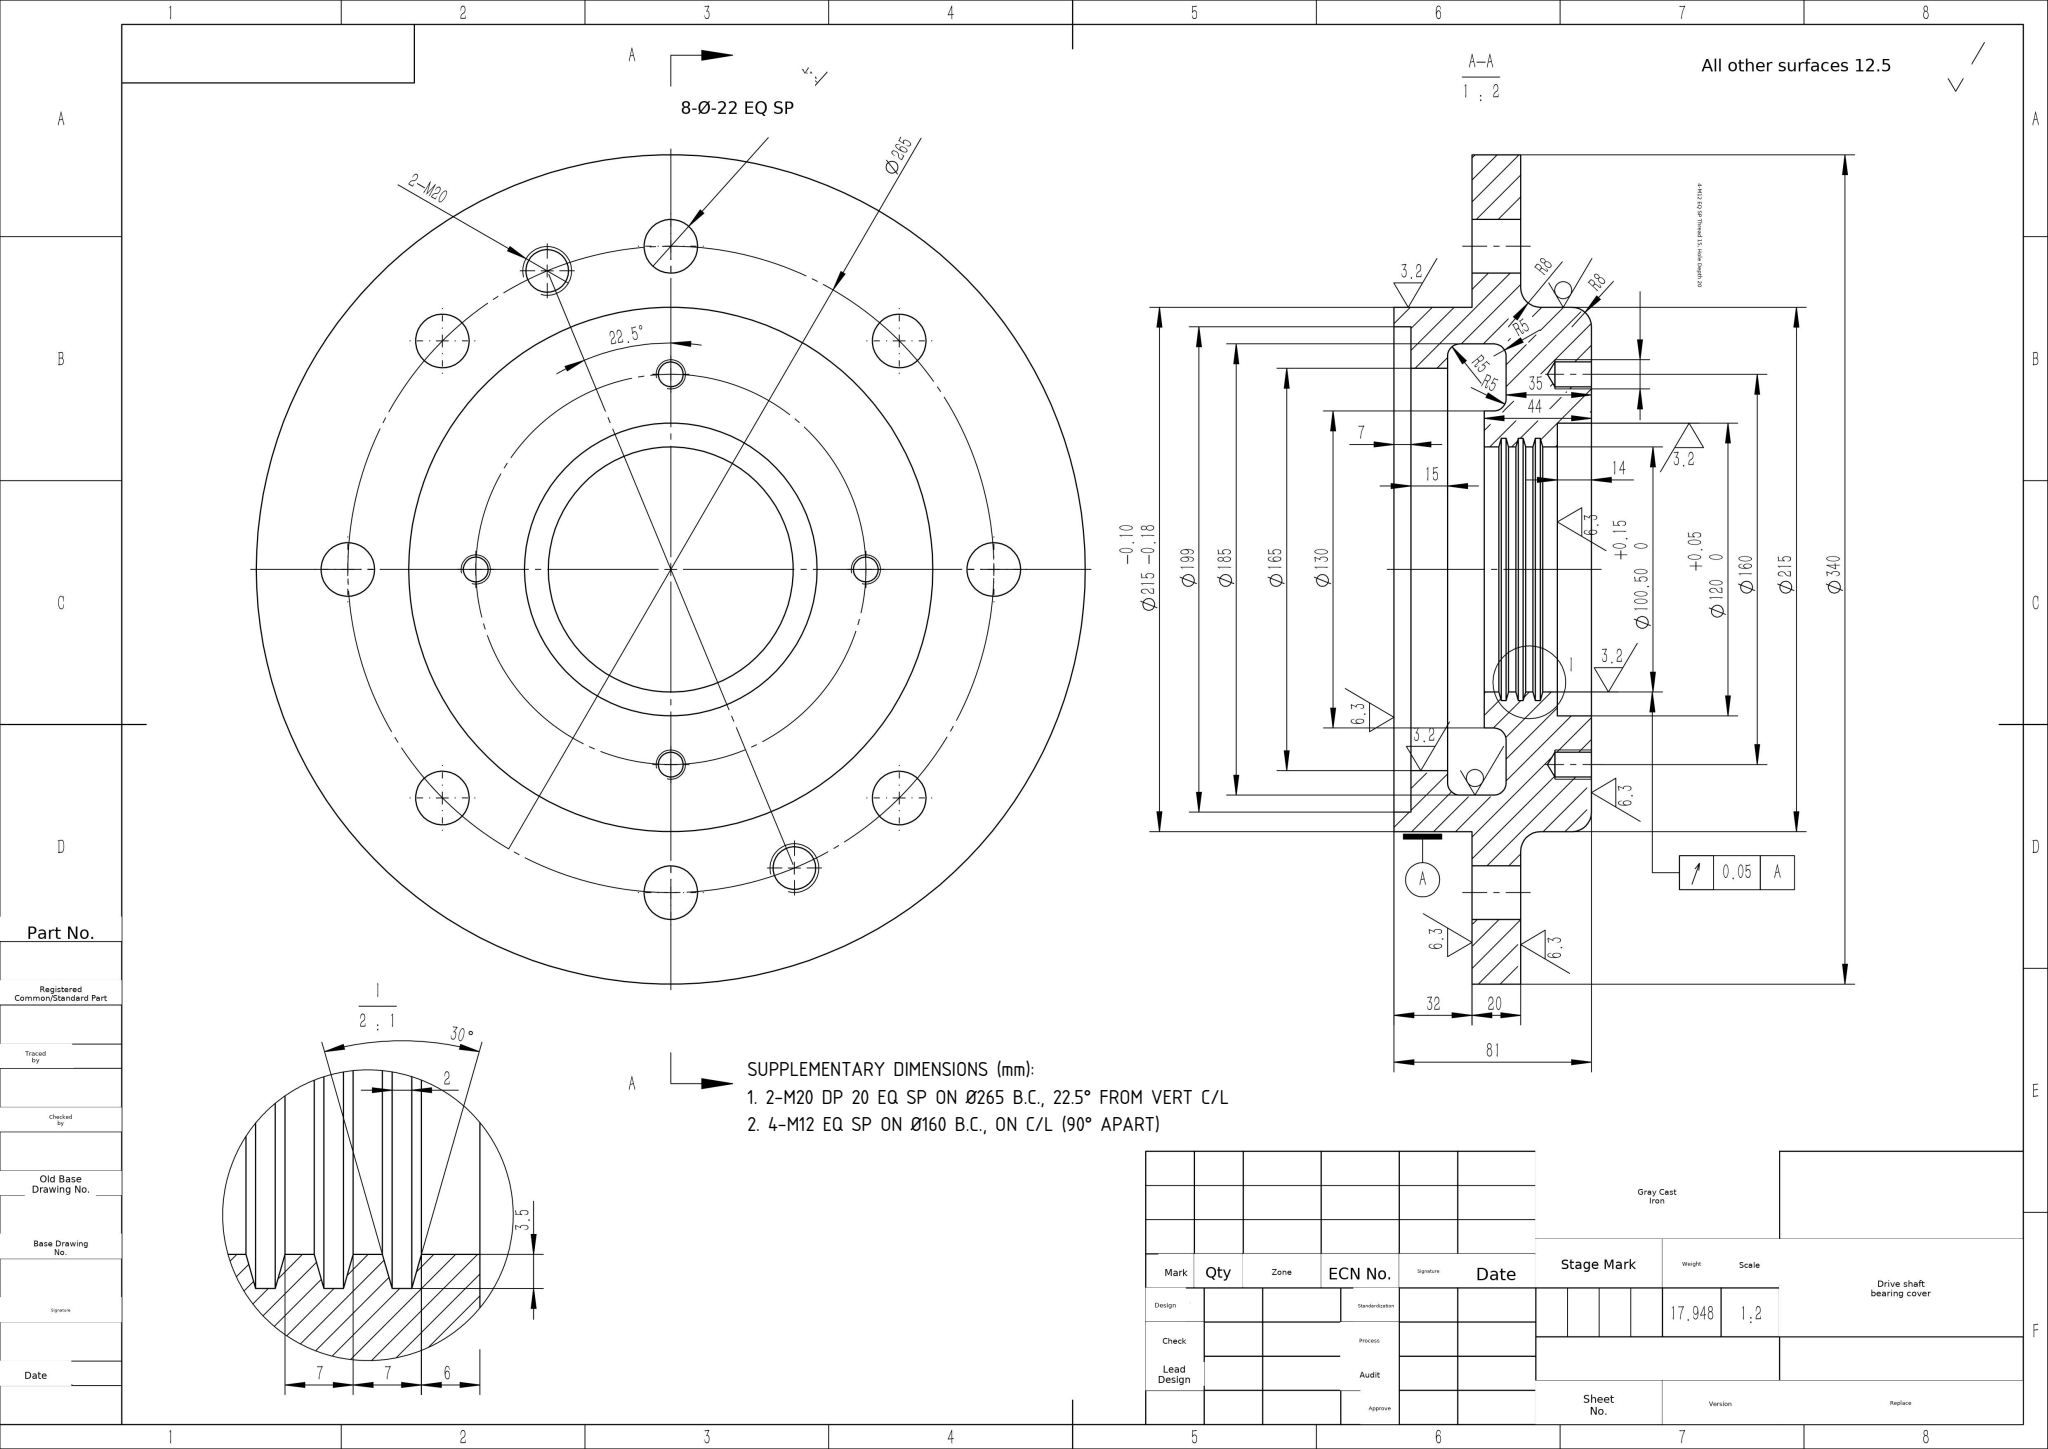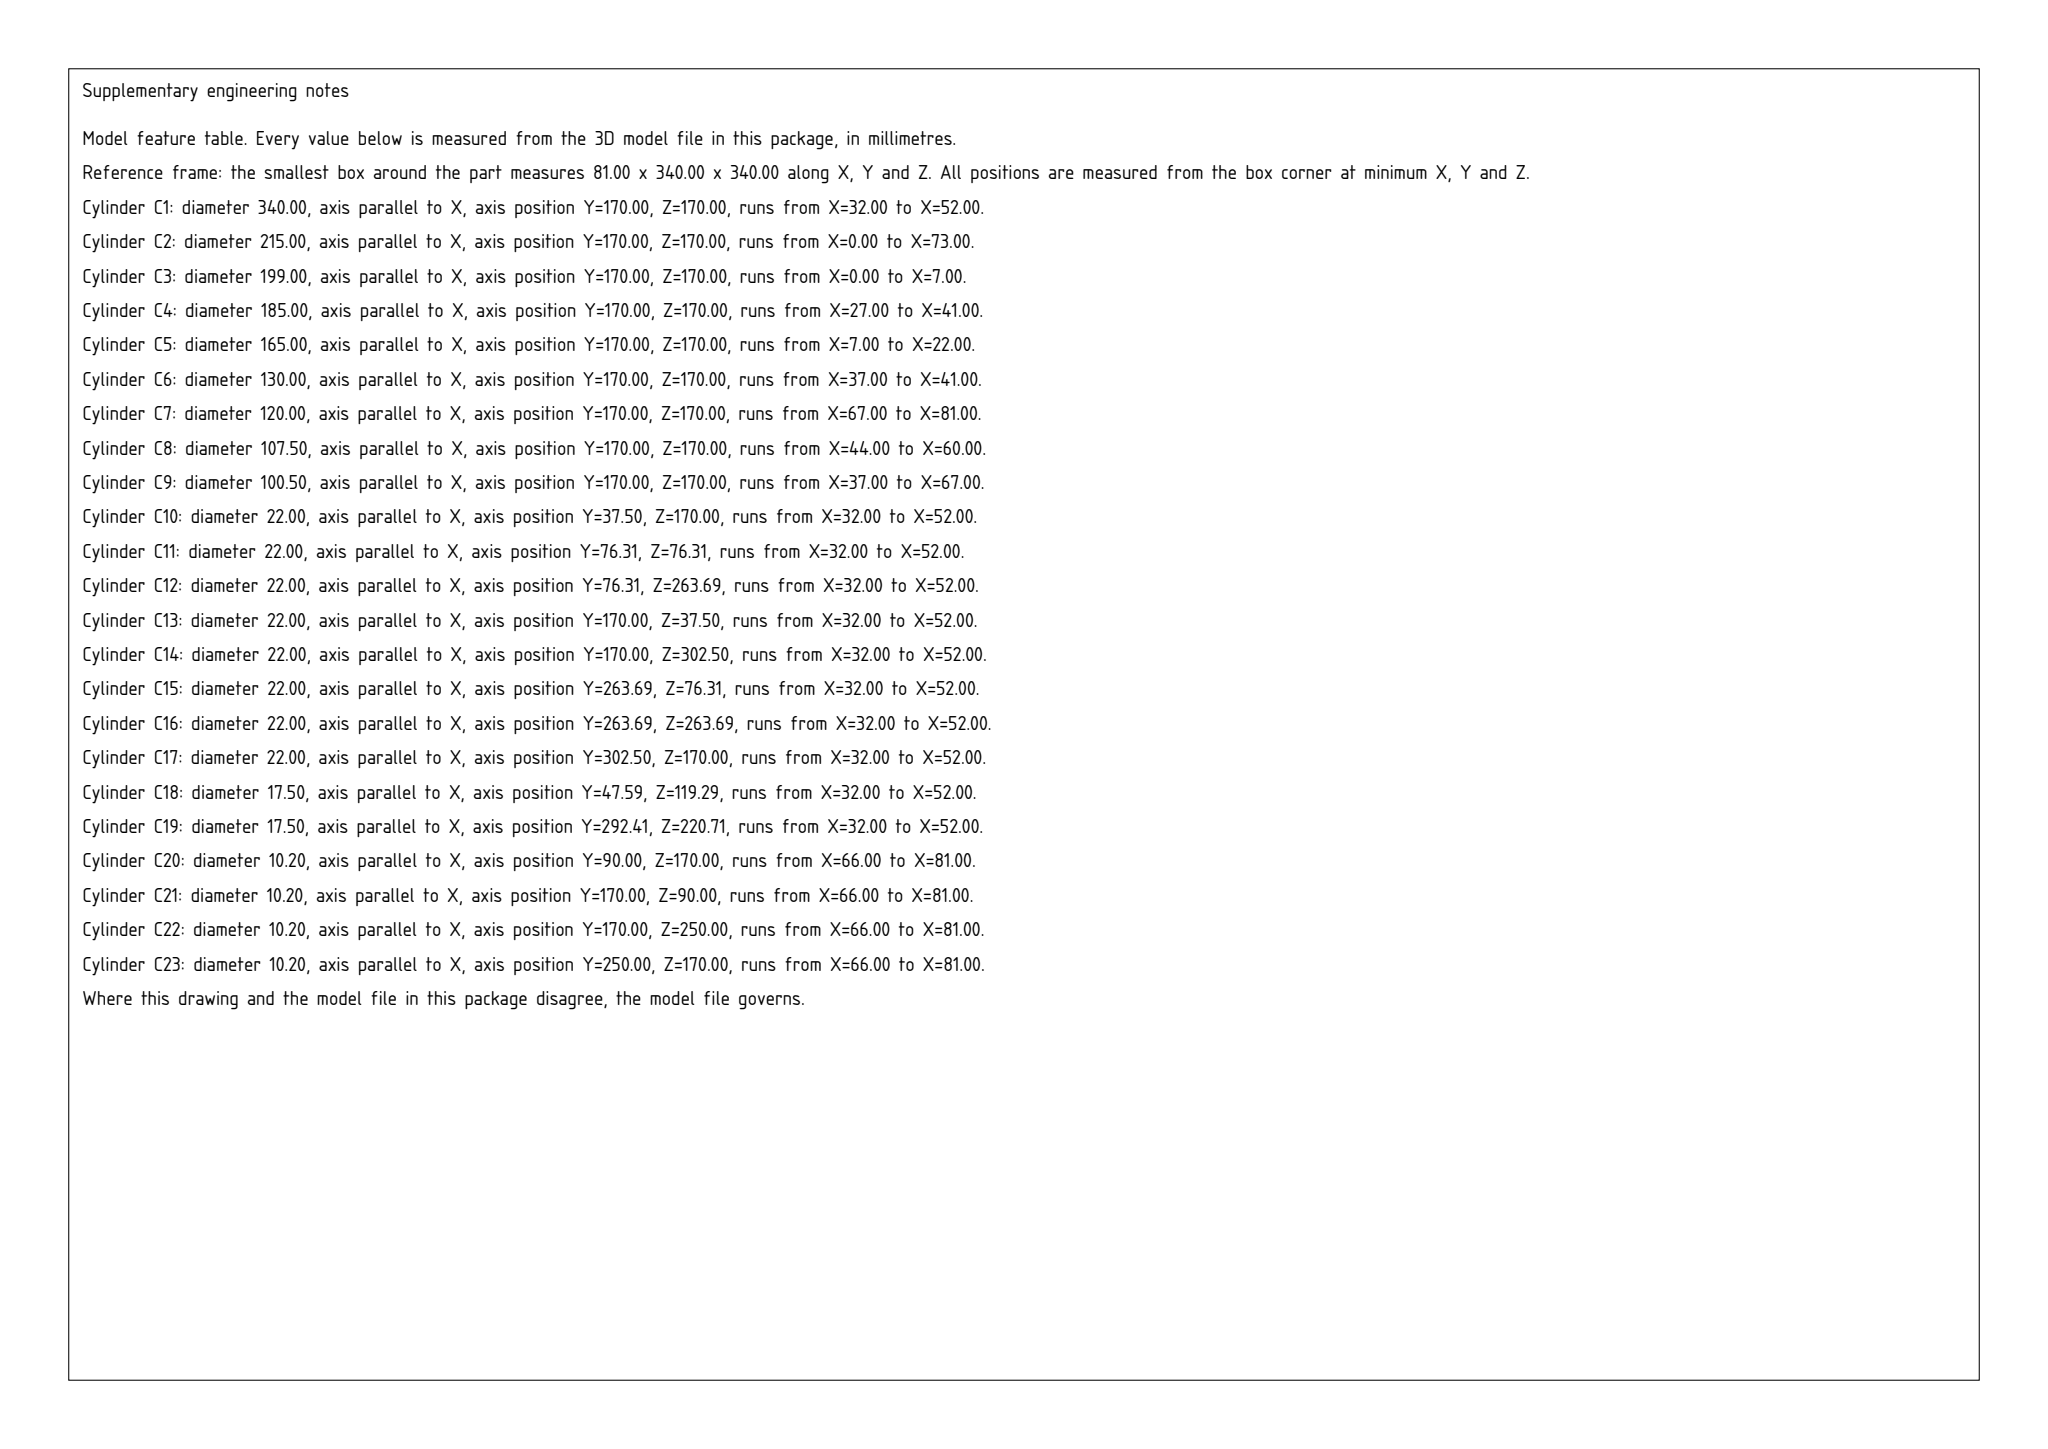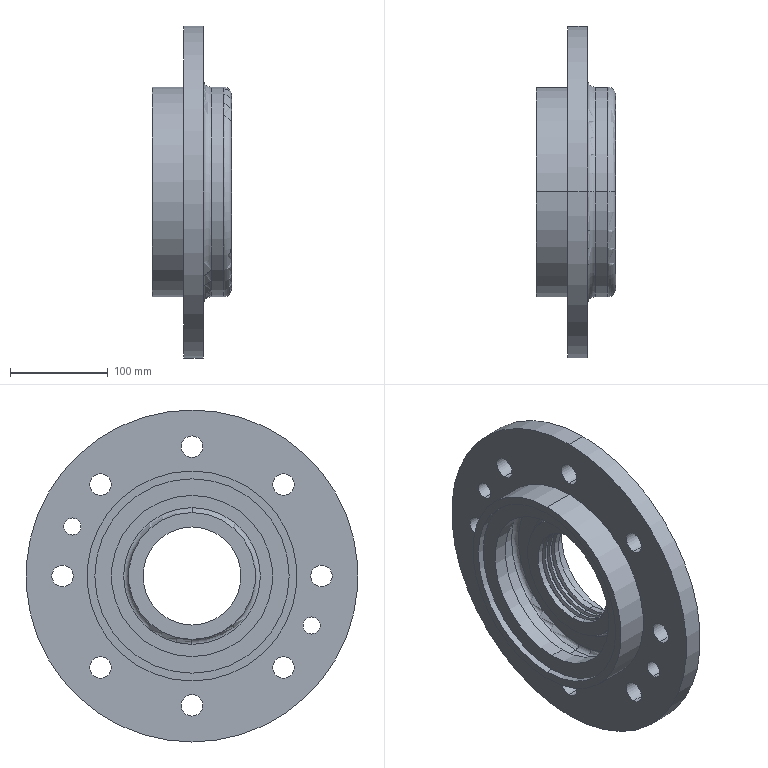Part | SolidWorks | mm | 1 solid | 97 faces | box 81 x 340 x 340 mm | volume 2492774 mm3 | cylinder 58 | cone 20 | torus 10 | plane 9 | commonest cylinder face diameters 22 x16 10.2 x8 100.5 x8 107.5 x6 17.5 x4 215 x4 185 x2 130 x2
build123d program:
from build123d import *

# Parameters (mm, degrees)
CUT_EXTRUDE1_REACH     = 247.976
SKETCH3_R              = 11
M20_TAPPED_HOLE1_D     = 17.5
M12_TAPPED_HOLE1_D     = 10.2
M12_TAPPED_HOLE1_DEPTH = 15
M12_TAPPED_HOLE1_TIP   = 3.064


with BuildPart() as part:
    # Sketch1 → Revolve1 (revolve)
    with BuildSketch(Plane.XY, mode=Mode.PRIVATE) as revolve1_sk:
        with BuildLine():
            Line((0, 82.5), (0, 99.5))
            Line((0, 99.5), (-7, 99.5))
            Line((-7, 99.5), (-7, 107.5))
            Line((-7, 107.5), (25, 107.5))
            Line((25, 107.5), (25, 170))
            Line((25, 170), (45, 170))
            Line((45, 170), (45, 115.5))
            ThreePointArc((45, 115.5), (47.343, 109.843), (53, 107.5))
            Line((53, 107.5), (66, 107.5))
            ThreePointArc((66, 107.5), (71.657, 105.157), (74, 99.5))
            Line((74, 99.5), (74, 60))
            Line((74, 60), (60, 60))
            Line((60, 60), (60, 50.25))
            Line((60, 50.25), (54, 50.25))
            Line((54, 50.25), (53, 53.75))
            Line((53, 53.75), (51, 53.75))
            Line((51, 53.75), (50, 50.25))
            Line((50, 50.25), (47, 50.25))
            Line((47, 50.25), (46, 53.75))
            Line((46, 53.75), (44, 53.75))
            Line((44, 53.75), (43, 50.25))
            Line((43, 50.25), (40, 50.25))
            Line((40, 50.25), (39, 53.75))
            Line((39, 53.75), (37, 53.75))
            Line((37, 53.75), (36, 50.25))
            Line((36, 50.25), (30, 50.25))
            Line((30, 50.25), (30, 65))
            Line((30, 65), (34, 65))
            ThreePointArc((34, 65), (37.536, 66.464), (39, 70))
            Line((39, 70), (39, 87.5))
            ThreePointArc((39, 87.5), (37.536, 91.036), (34, 92.5))
            Line((34, 92.5), (20, 92.5))
            ThreePointArc((20, 92.5), (16.464, 91.036), (15, 87.5))
            Line((15, 87.5), (15, 82.5))
            Line((15, 82.5), (0, 82.5))
        make_face()
    revolve(revolve1_sk.sketch.rotate(Axis((0, 0, 0), (1, 0, 0)), 90), axis=Axis((0, 0, 0), (1, 0, 0)))

    # Sketch3 → Cut-Extrude1 (cut, up to next)
    with BuildSketch(Plane(origin=(45, 0, 0), x_dir=(0, 0, -1), z_dir=(1, 0, 0)), mode=Mode.PRIVATE) as cut_extrude1_sk1:
        with Locations((0, 132.5)):
            Circle(SKETCH3_R)
    cut_extrude1_tool1 = extrude(cut_extrude1_sk1.sketch, amount=-CUT_EXTRUDE1_REACH, mode=Mode.PRIVATE) & part.part
    # Sketch3 → Cut-Extrude1 (cut, up to next)
    with BuildSketch(Plane(origin=(45, 0, 0), x_dir=(0, 0, -1), z_dir=(1, 0, 0)), mode=Mode.PRIVATE) as cut_extrude1_sk2:
        with Locations((93.692, 93.692)):
            Circle(SKETCH3_R)
    cut_extrude1_tool2 = extrude(cut_extrude1_sk2.sketch, amount=-CUT_EXTRUDE1_REACH, mode=Mode.PRIVATE) & part.part
    # Sketch3 → Cut-Extrude1 (cut, up to next)
    with BuildSketch(Plane(origin=(45, 0, 0), x_dir=(0, 0, -1), z_dir=(1, 0, 0)), mode=Mode.PRIVATE) as cut_extrude1_sk3:
        with Locations((132.5, 0)):
            Circle(SKETCH3_R)
    cut_extrude1_tool3 = extrude(cut_extrude1_sk3.sketch, amount=-CUT_EXTRUDE1_REACH, mode=Mode.PRIVATE) & part.part
    # Sketch3 → Cut-Extrude1 (cut, up to next)
    with BuildSketch(Plane(origin=(45, 0, 0), x_dir=(0, 0, -1), z_dir=(1, 0, 0)), mode=Mode.PRIVATE) as cut_extrude1_sk4:
        with Locations((93.692, -93.692)):
            Circle(SKETCH3_R)
    cut_extrude1_tool4 = extrude(cut_extrude1_sk4.sketch, amount=-CUT_EXTRUDE1_REACH, mode=Mode.PRIVATE) & part.part
    # Sketch3 → Cut-Extrude1 (cut, up to next)
    with BuildSketch(Plane(origin=(45, 0, 0), x_dir=(0, 0, -1), z_dir=(1, 0, 0)), mode=Mode.PRIVATE) as cut_extrude1_sk5:
        with Locations((0, -132.5)):
            Circle(SKETCH3_R)
    cut_extrude1_tool5 = extrude(cut_extrude1_sk5.sketch, amount=-CUT_EXTRUDE1_REACH, mode=Mode.PRIVATE) & part.part
    # Sketch3 → Cut-Extrude1 (cut, up to next)
    with BuildSketch(Plane(origin=(45, 0, 0), x_dir=(0, 0, -1), z_dir=(1, 0, 0)), mode=Mode.PRIVATE) as cut_extrude1_sk6:
        with Locations((-93.692, -93.692)):
            Circle(SKETCH3_R)
    cut_extrude1_tool6 = extrude(cut_extrude1_sk6.sketch, amount=-CUT_EXTRUDE1_REACH, mode=Mode.PRIVATE) & part.part
    # Sketch3 → Cut-Extrude1 (cut, up to next)
    with BuildSketch(Plane(origin=(45, 0, 0), x_dir=(0, 0, -1), z_dir=(1, 0, 0)), mode=Mode.PRIVATE) as cut_extrude1_sk7:
        with Locations((-132.5, 0)):
            Circle(SKETCH3_R)
    cut_extrude1_tool7 = extrude(cut_extrude1_sk7.sketch, amount=-CUT_EXTRUDE1_REACH, mode=Mode.PRIVATE) & part.part
    # Sketch3 → Cut-Extrude1 (cut, up to next)
    with BuildSketch(Plane(origin=(45, 0, 0), x_dir=(0, 0, -1), z_dir=(1, 0, 0)), mode=Mode.PRIVATE) as cut_extrude1_sk8:
        with Locations((-93.692, 93.692)):
            Circle(SKETCH3_R)
    cut_extrude1_tool8 = extrude(cut_extrude1_sk8.sketch, amount=-CUT_EXTRUDE1_REACH, mode=Mode.PRIVATE) & part.part
    add(cut_extrude1_tool1.solids().sort_by_distance((45, 132.5, 0))[0], mode=Mode.SUBTRACT)
    add(cut_extrude1_tool2.solids().sort_by_distance((45, 93.692, -93.692))[0], mode=Mode.SUBTRACT)
    add(cut_extrude1_tool3.solids().sort_by_distance((45, 0, -132.5))[0], mode=Mode.SUBTRACT)
    add(cut_extrude1_tool4.solids().sort_by_distance((45, -93.692, -93.692))[0], mode=Mode.SUBTRACT)
    add(cut_extrude1_tool5.solids().sort_by_distance((45, -132.5, 0))[0], mode=Mode.SUBTRACT)
    add(cut_extrude1_tool6.solids().sort_by_distance((45, -93.692, 93.692))[0], mode=Mode.SUBTRACT)
    add(cut_extrude1_tool7.solids().sort_by_distance((45, 0, 132.5))[0], mode=Mode.SUBTRACT)
    add(cut_extrude1_tool8.solids().sort_by_distance((45, 93.692, 93.692))[0], mode=Mode.SUBTRACT)

    # M20 Tapped Hole1 (through all)
    with Locations(Plane(origin=(45, -122.414, -50.706), x_dir=(0, 0, 1), z_dir=(1, 0, 0))):
        with Locations((0, 0), (101.411, -244.828)):
            Hole(M20_TAPPED_HOLE1_D / 2)

    # M12 Tapped Hole1
    with Locations(Plane(origin=(74, 80, 0), x_dir=(0, 0, 1), z_dir=(1, 0, 0))):
        with Locations((0, 0), (-80, 80), (0, 160), (80, 80)):
            Hole(M12_TAPPED_HOLE1_D / 2, depth=M12_TAPPED_HOLE1_DEPTH)
            with Locations((0, 0, -(M12_TAPPED_HOLE1_DEPTH + M12_TAPPED_HOLE1_TIP / 2))):  # 118° drill point
                Cone(0, M12_TAPPED_HOLE1_D / 2, M12_TAPPED_HOLE1_TIP, mode=Mode.SUBTRACT)


solid = part.part